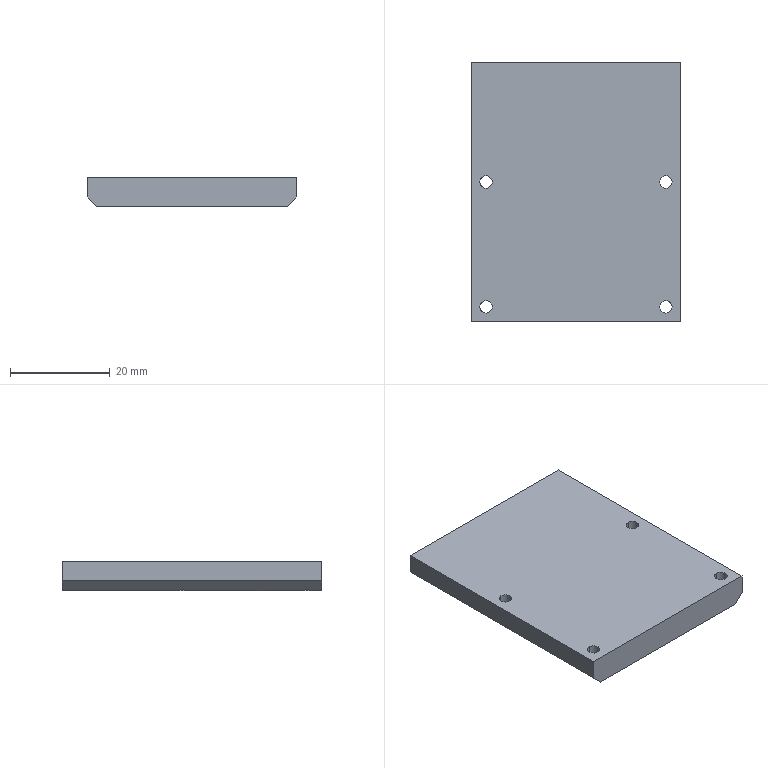CAM job | Mastercam | mm | 8 operations | part box 42 x 52 x 6
1. Facing | 24 - 100 平铣刀
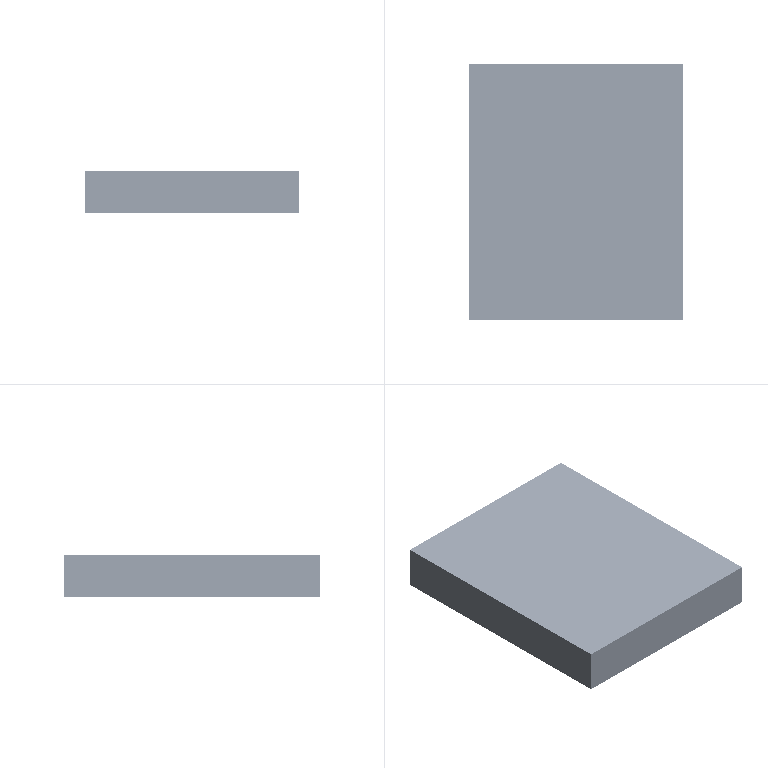2. Contour (Ramp) | 10 - 10 平铣刀
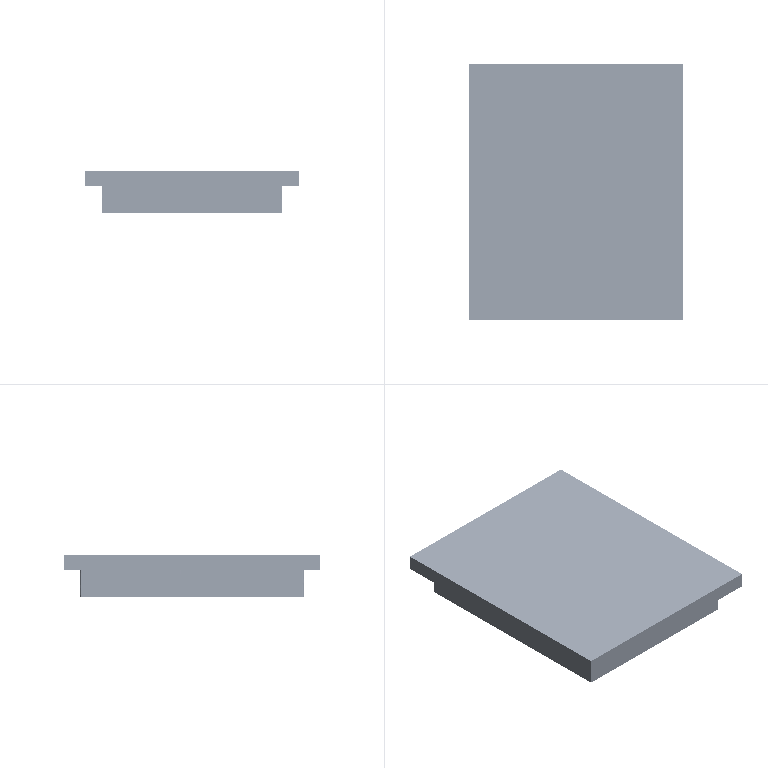3. Contour (2D) | 10 - 10 平铣刀
4. Surface Finish Flowline | 10 - 10 平铣刀
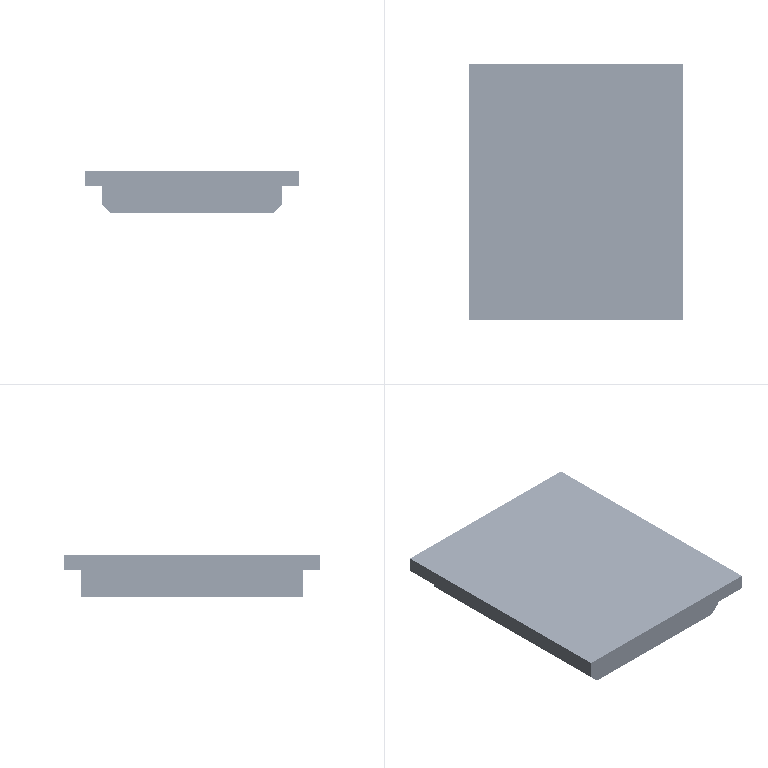5. Facing | 24 - 100 平铣刀
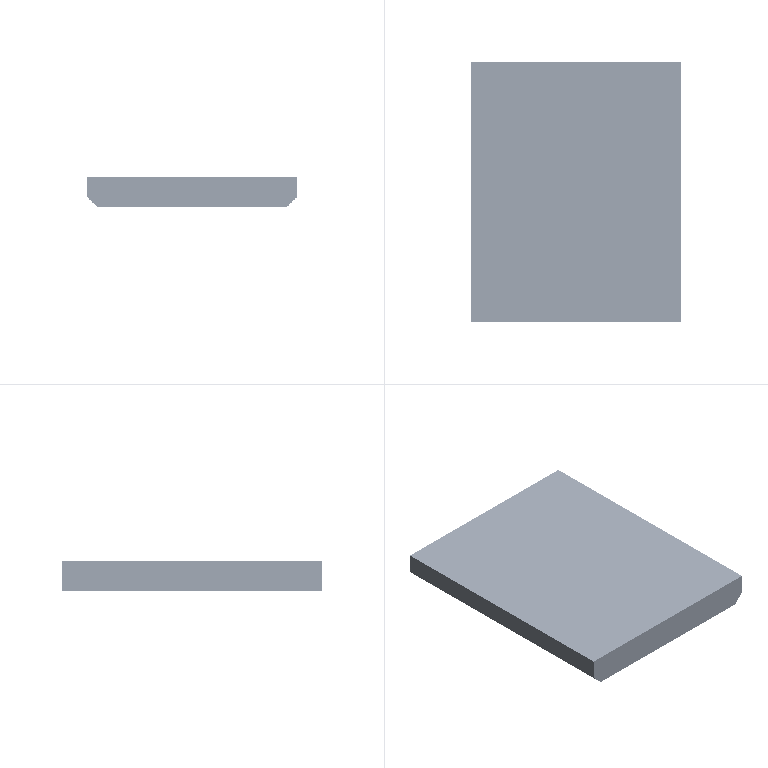6. Drill/Counterbore | 7 - 4 倒角刀
7. Contour (2D chamfer) | 7 - 4 倒角刀
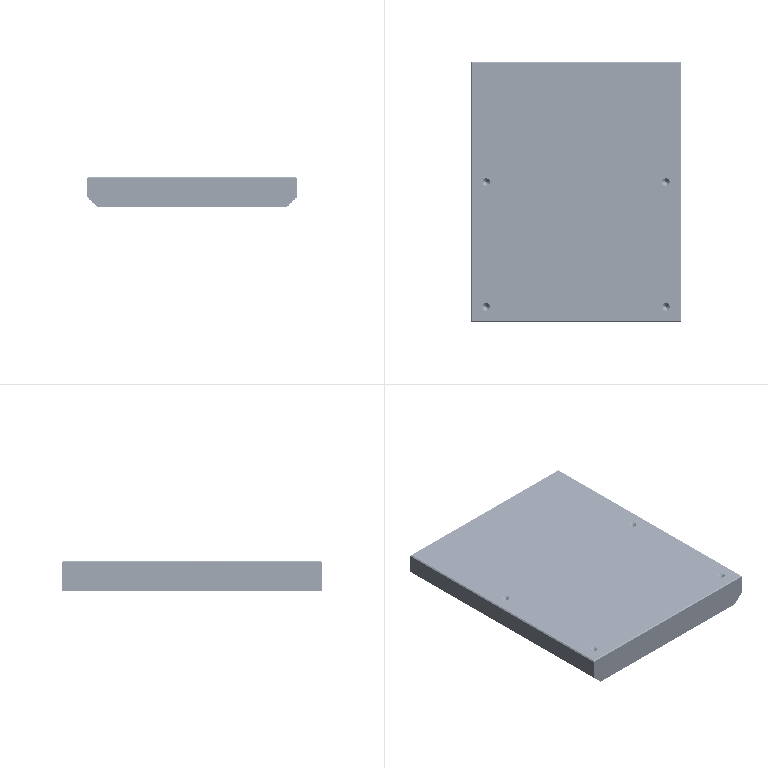8. Drill/Counterbore | 7 - 4 倒角刀